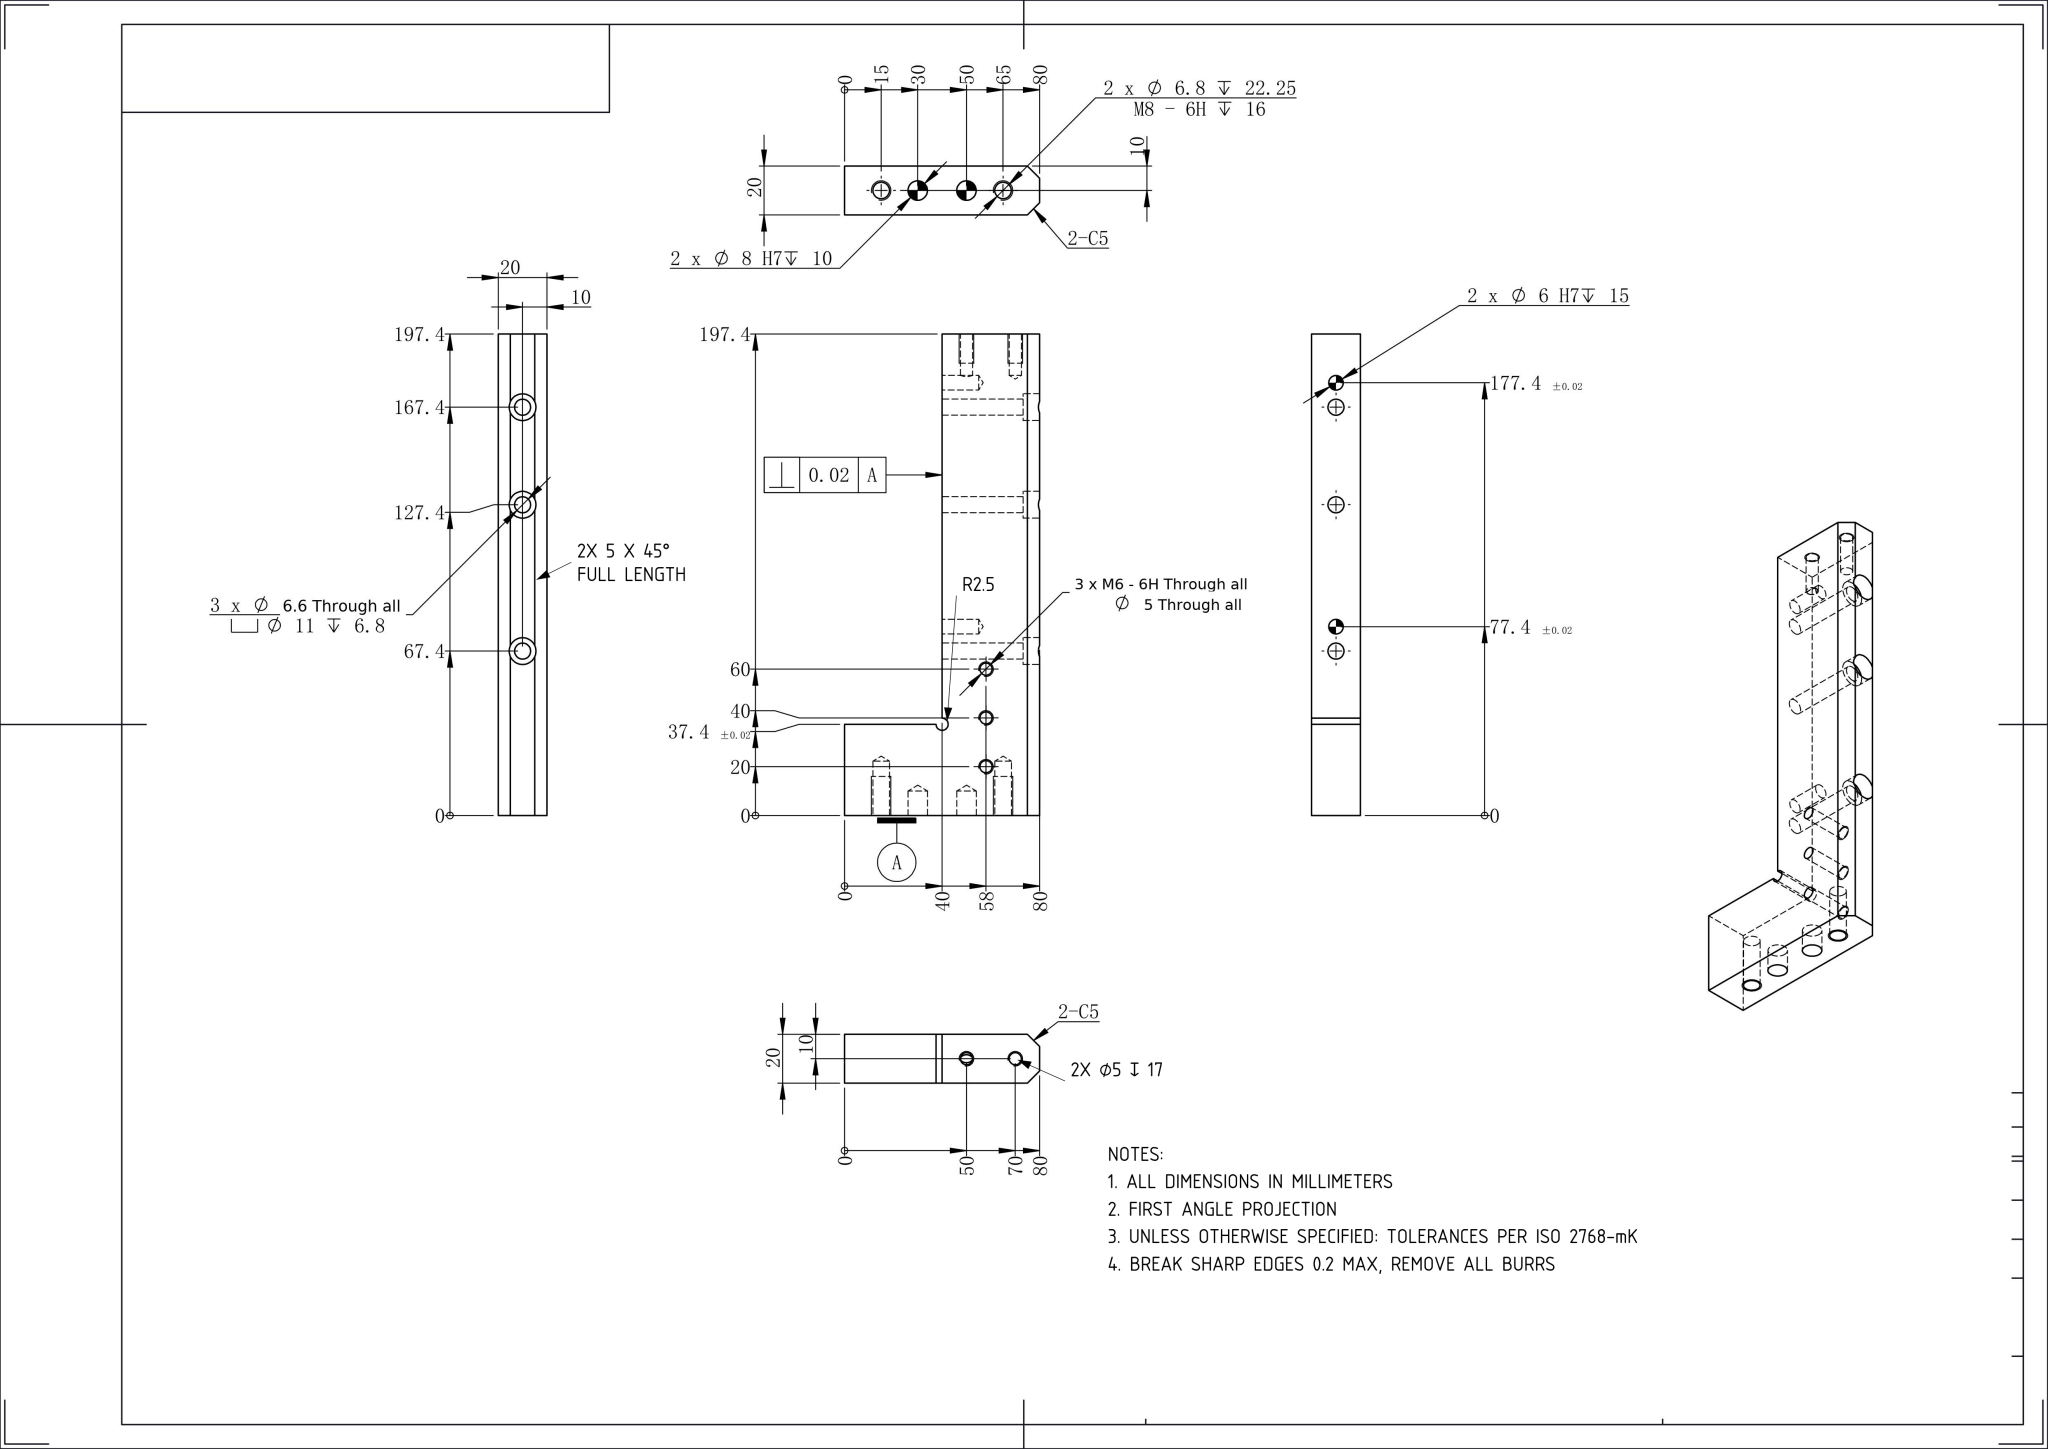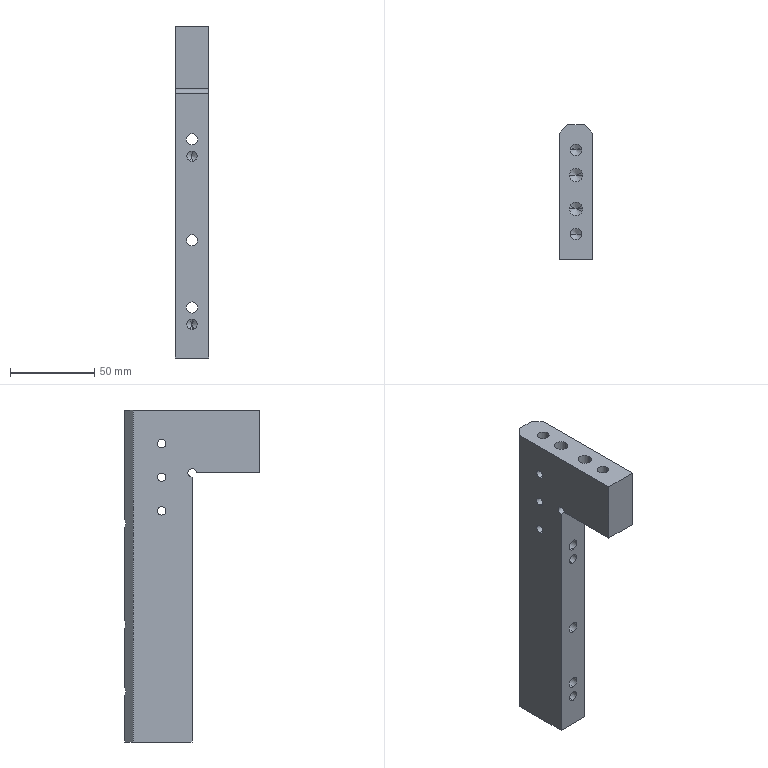Part | NX | mm | 1 solid | 67 faces | box 20 x 80 x 197.4 mm | volume 171774 mm3 | cylinder 35 | cone 16 | plane 16 | commonest cylinder face diameters 5 x11 11 x6 6.6 x6 8 x4 6.8 x4 6 x4